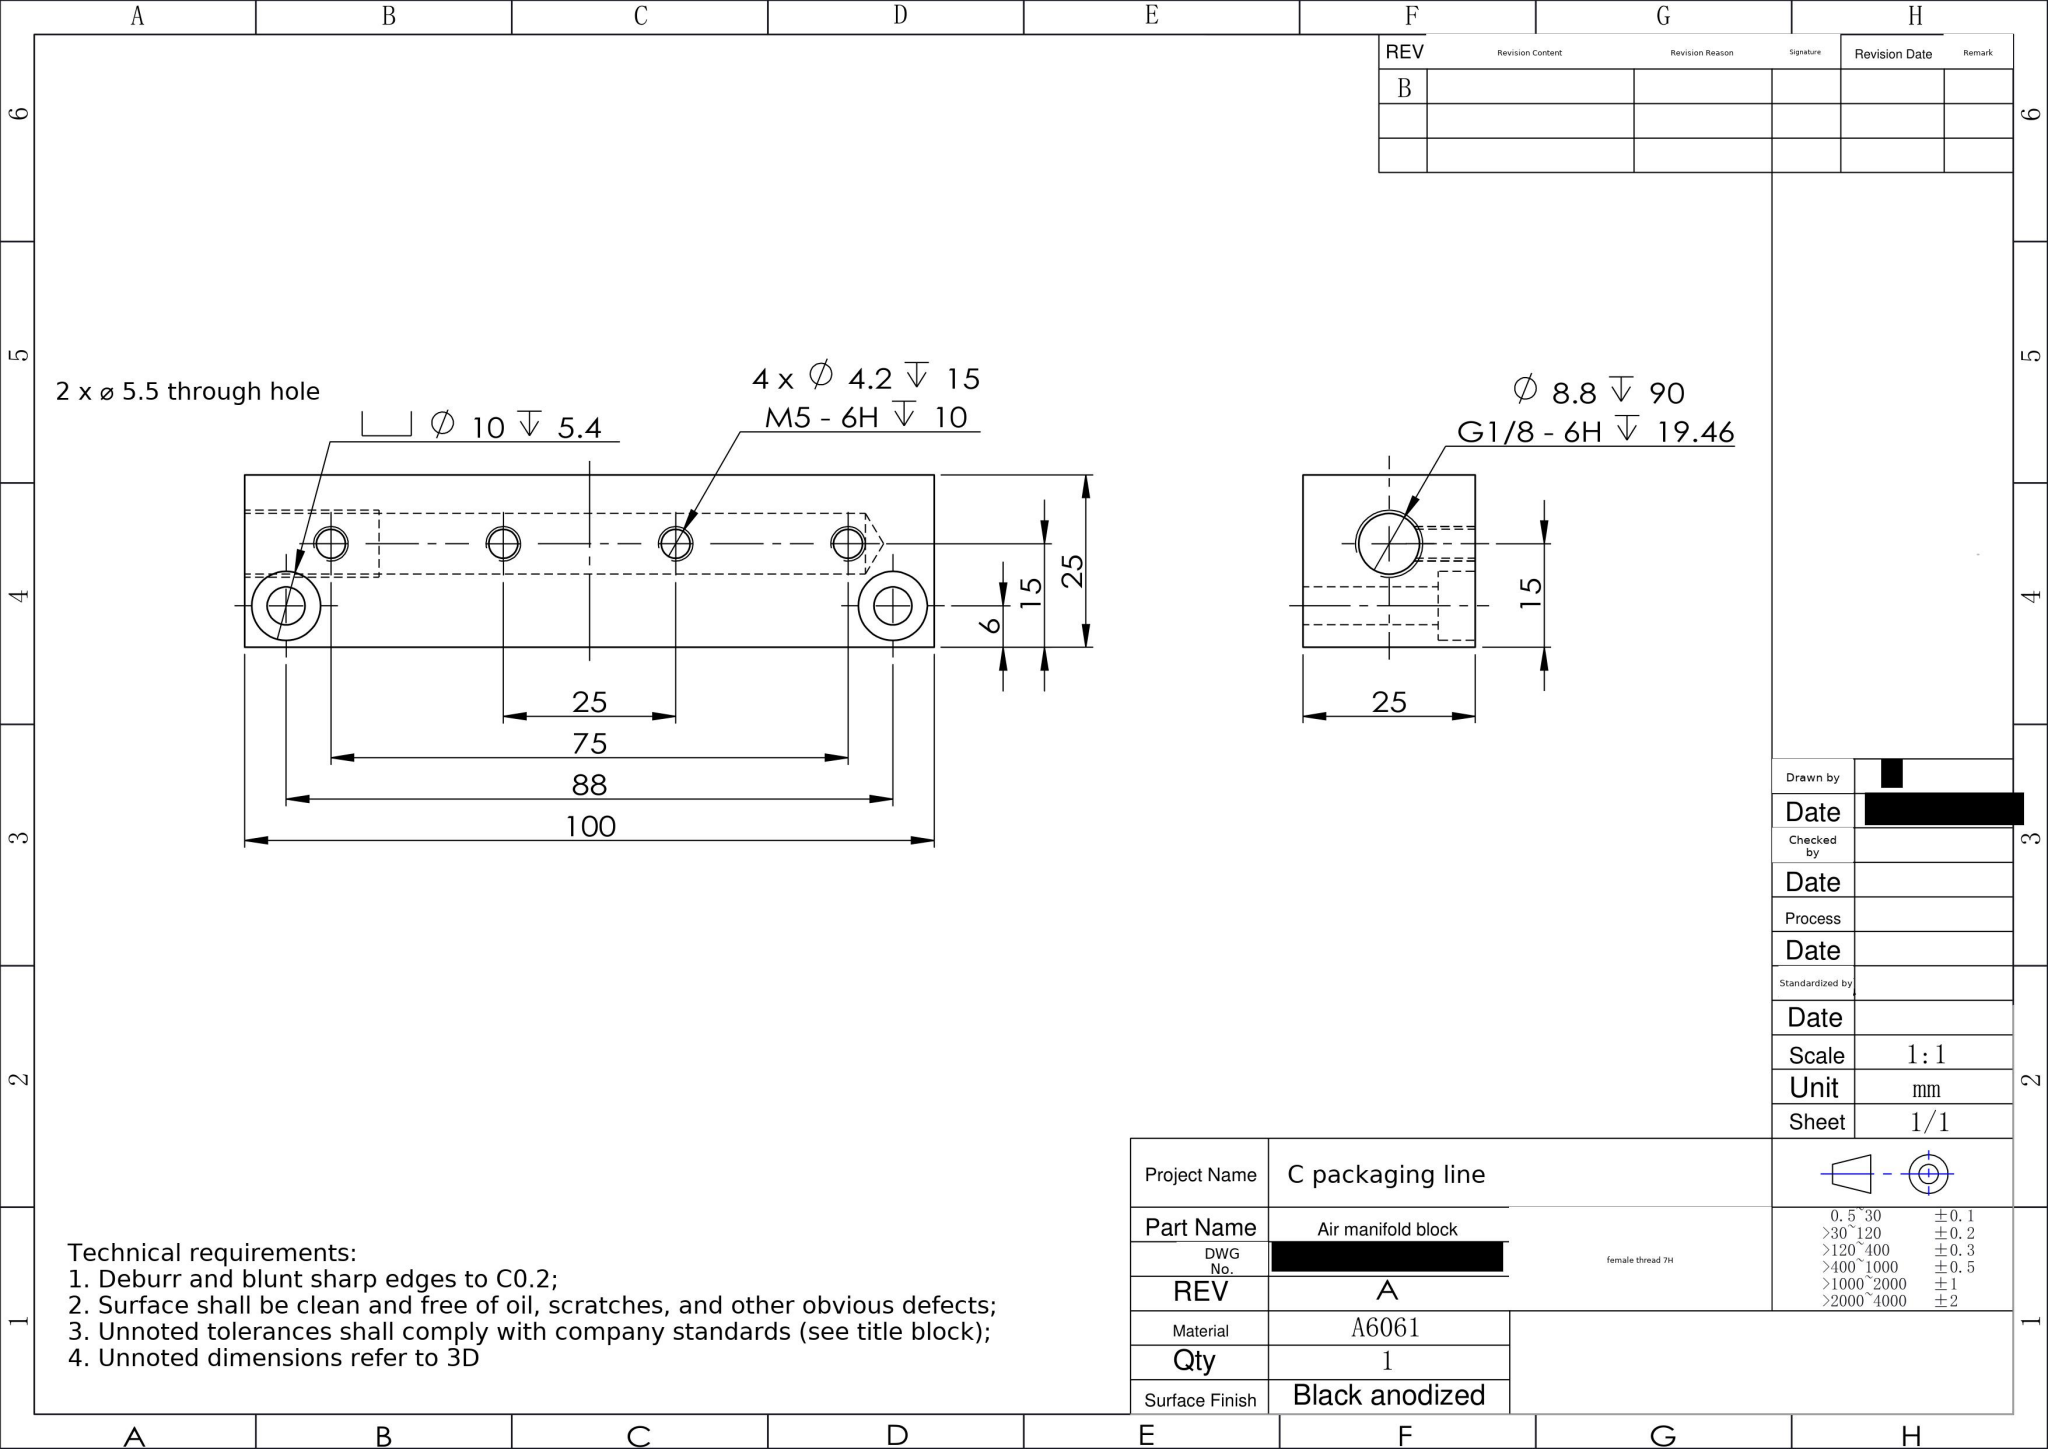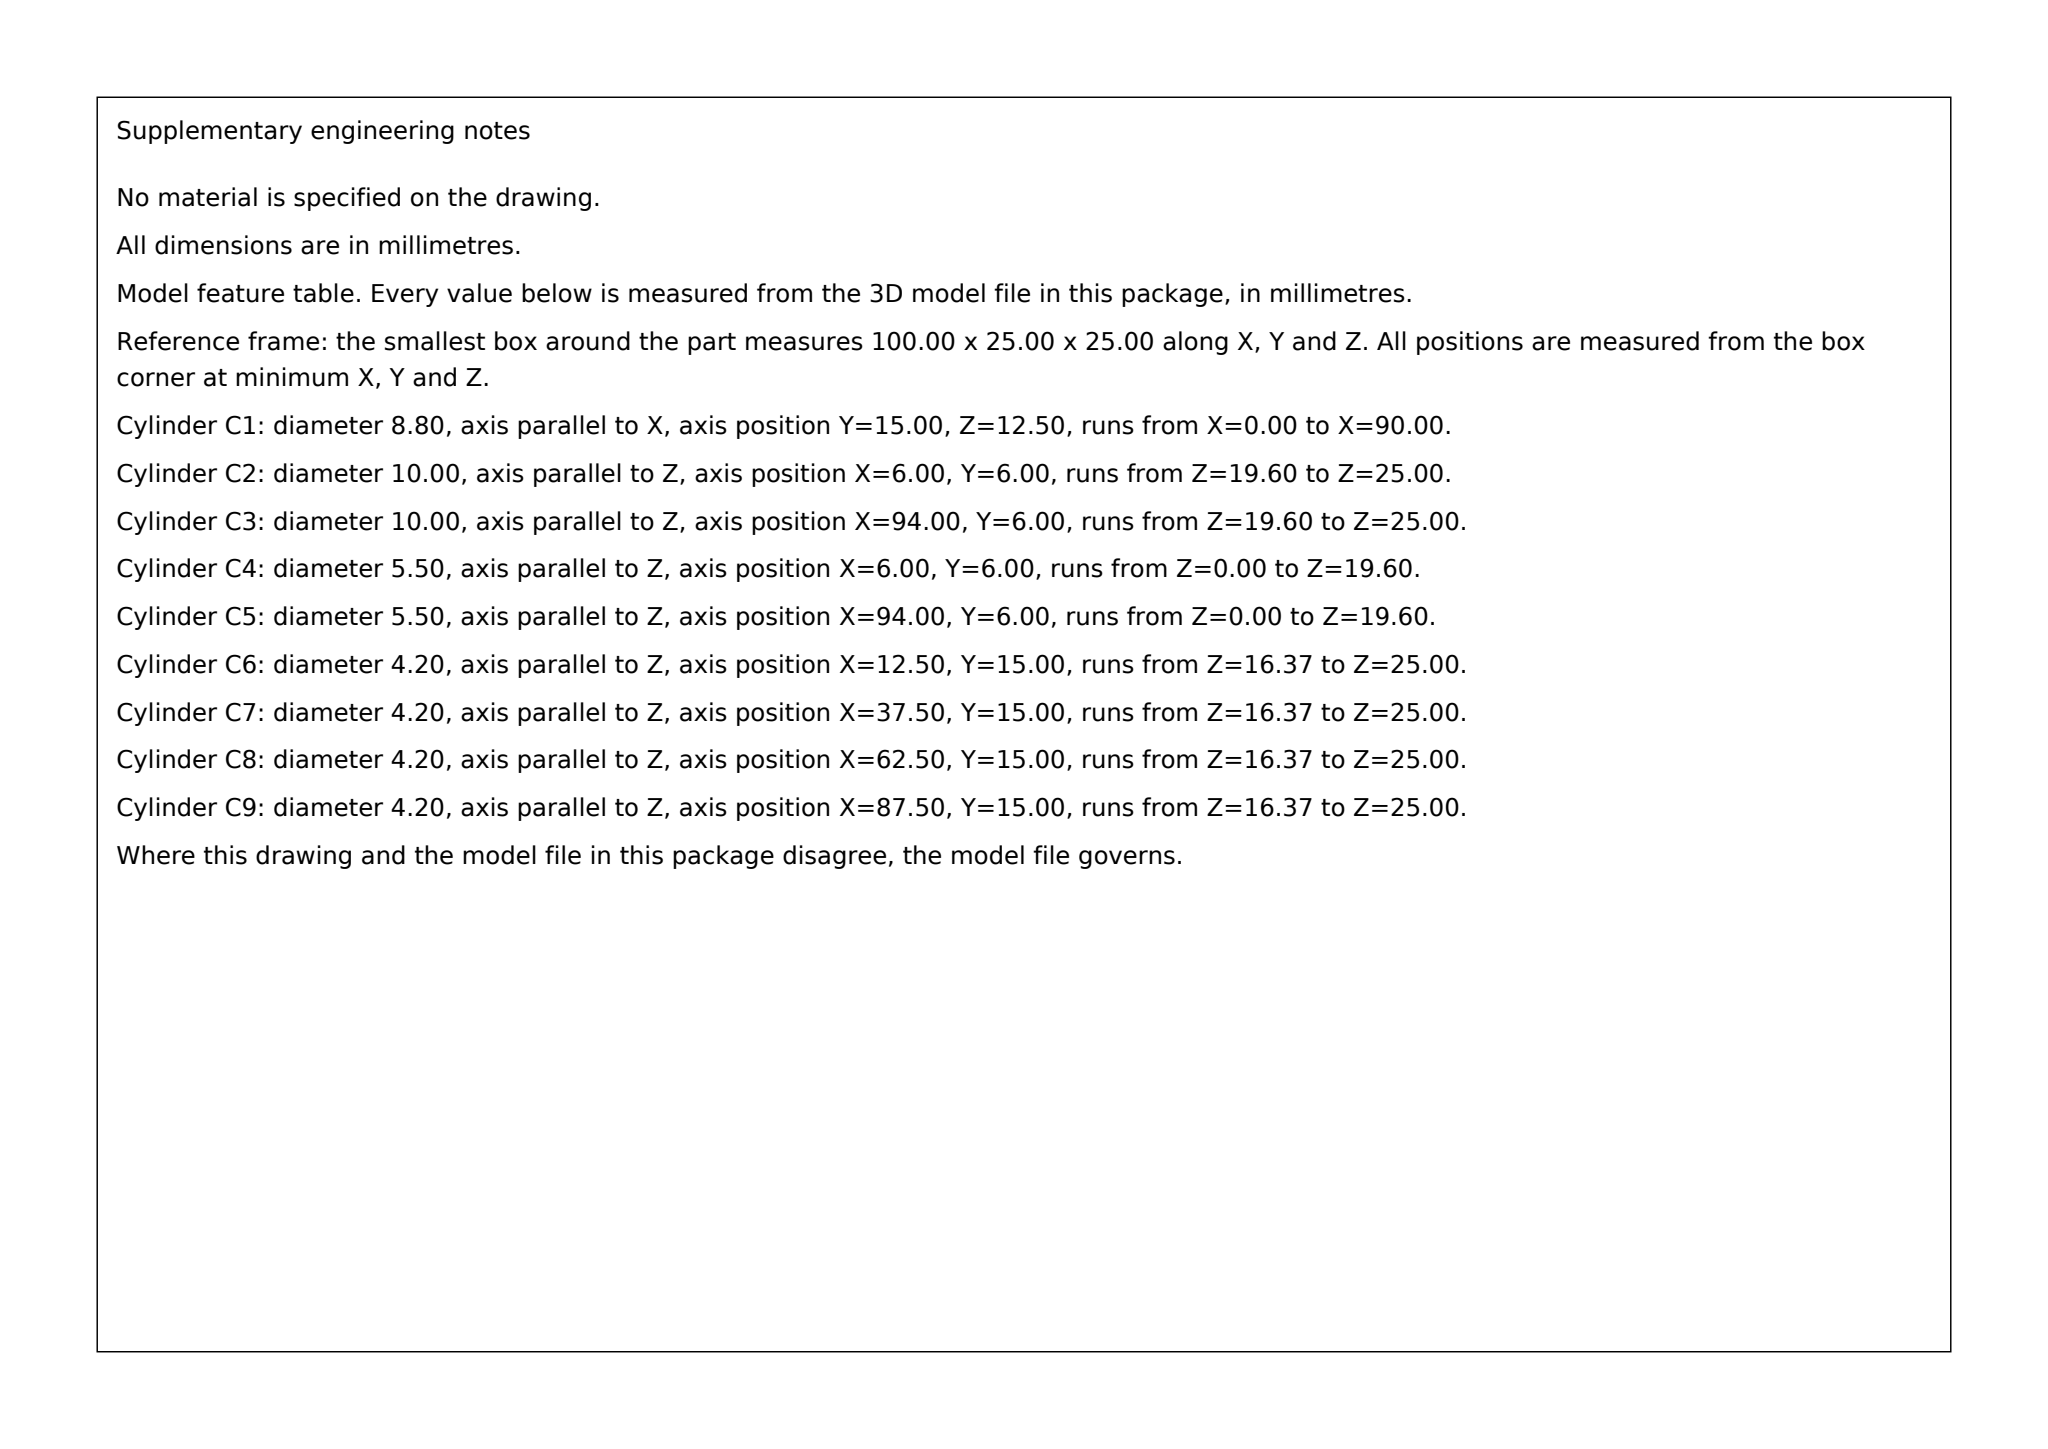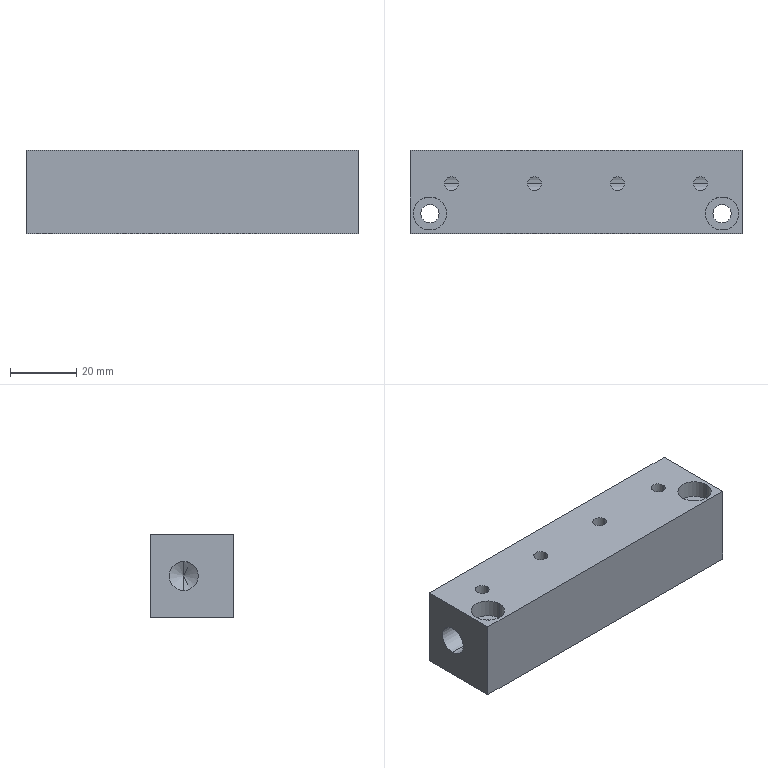Part | SolidWorks | mm | 1 solid | 28 faces | box 100 x 25 x 25 mm | volume 54737 mm3 | cylinder 18 | plane 8 | cone 2 | commonest cylinder face diameters 4.2 x8 10 x4 5.5 x4 8.8 x2
build123d program:
from build123d import *

# Parameters (mm, degrees)
SKETCH1_W                                       = 100
SKETCH1_H                                       = 25
BOSS_EXTRUDE1_DEPTH                             = 25
LPATTERN1_COUNT                                 = 4
LPATTERN1_PITCH                                 = 25
M5_HEX_SOCKET_HEAD_CAP_SCREW_CBORE1_D           = 5.5
M5_HEX_SOCKET_HEAD_CAP_SCREW_CBORE1_CBORE_D     = 10
M5_HEX_SOCKET_HEAD_CAP_SCREW_CBORE1_CBORE_DEPTH = 5.4
G1_8_TAPPED_HOLE2_D                             = 8.8
G1_8_TAPPED_HOLE2_DEPTH                         = 90
G1_8_TAPPED_HOLE2_TIP                           = 2.644


with BuildPart() as part:
    # Sketch1 → Boss-Extrude1 (new body)
    with BuildSketch(Plane.XY):
        Rectangle(SKETCH1_W, SKETCH1_H)
    extrude(amount=BOSS_EXTRUDE1_DEPTH)

    # Sketch3 → M5 Tapped Hole1 (revolve, cut)
    with BuildSketch(Plane(origin=(-37.5, 2.5, 25), x_dir=(0, -1, 0), z_dir=(1, 0, 0))):
        Polygon((0, 0), (0, 16.262), (2.1, 15), (2.1, 0), align=None)
    m5_tapped_hole1 = revolve(axis=Axis((-37.5, 2.5, 31.35), (0, 0, -1)), mode=Mode.SUBTRACT)

    # LPattern1: M5 Tapped Hole1 ×4
    with Locations(*[(i * LPATTERN1_PITCH, 0, 0) for i in range(1, LPATTERN1_COUNT)]):
        add(m5_tapped_hole1, mode=Mode.SUBTRACT)

    # M5 Hex Socket Head Cap Screw CBORE1 (through all)
    with Locations(Plane.XY.offset(25)):
        with Locations((-44, -6.5), (44, -6.5)):
            CounterBoreHole(M5_HEX_SOCKET_HEAD_CAP_SCREW_CBORE1_D / 2, M5_HEX_SOCKET_HEAD_CAP_SCREW_CBORE1_CBORE_D / 2, M5_HEX_SOCKET_HEAD_CAP_SCREW_CBORE1_CBORE_DEPTH)

    # G1_8 Tapped Hole2
    with Locations(Plane.ZY.offset(50)):
        with Locations((12.5, 2.5)):
            Hole(G1_8_TAPPED_HOLE2_D / 2, depth=G1_8_TAPPED_HOLE2_DEPTH)
            with Locations((0, 0, -(G1_8_TAPPED_HOLE2_DEPTH + G1_8_TAPPED_HOLE2_TIP / 2))):  # 118° drill point
                Cone(0, G1_8_TAPPED_HOLE2_D / 2, G1_8_TAPPED_HOLE2_TIP, mode=Mode.SUBTRACT)


solid = part.part